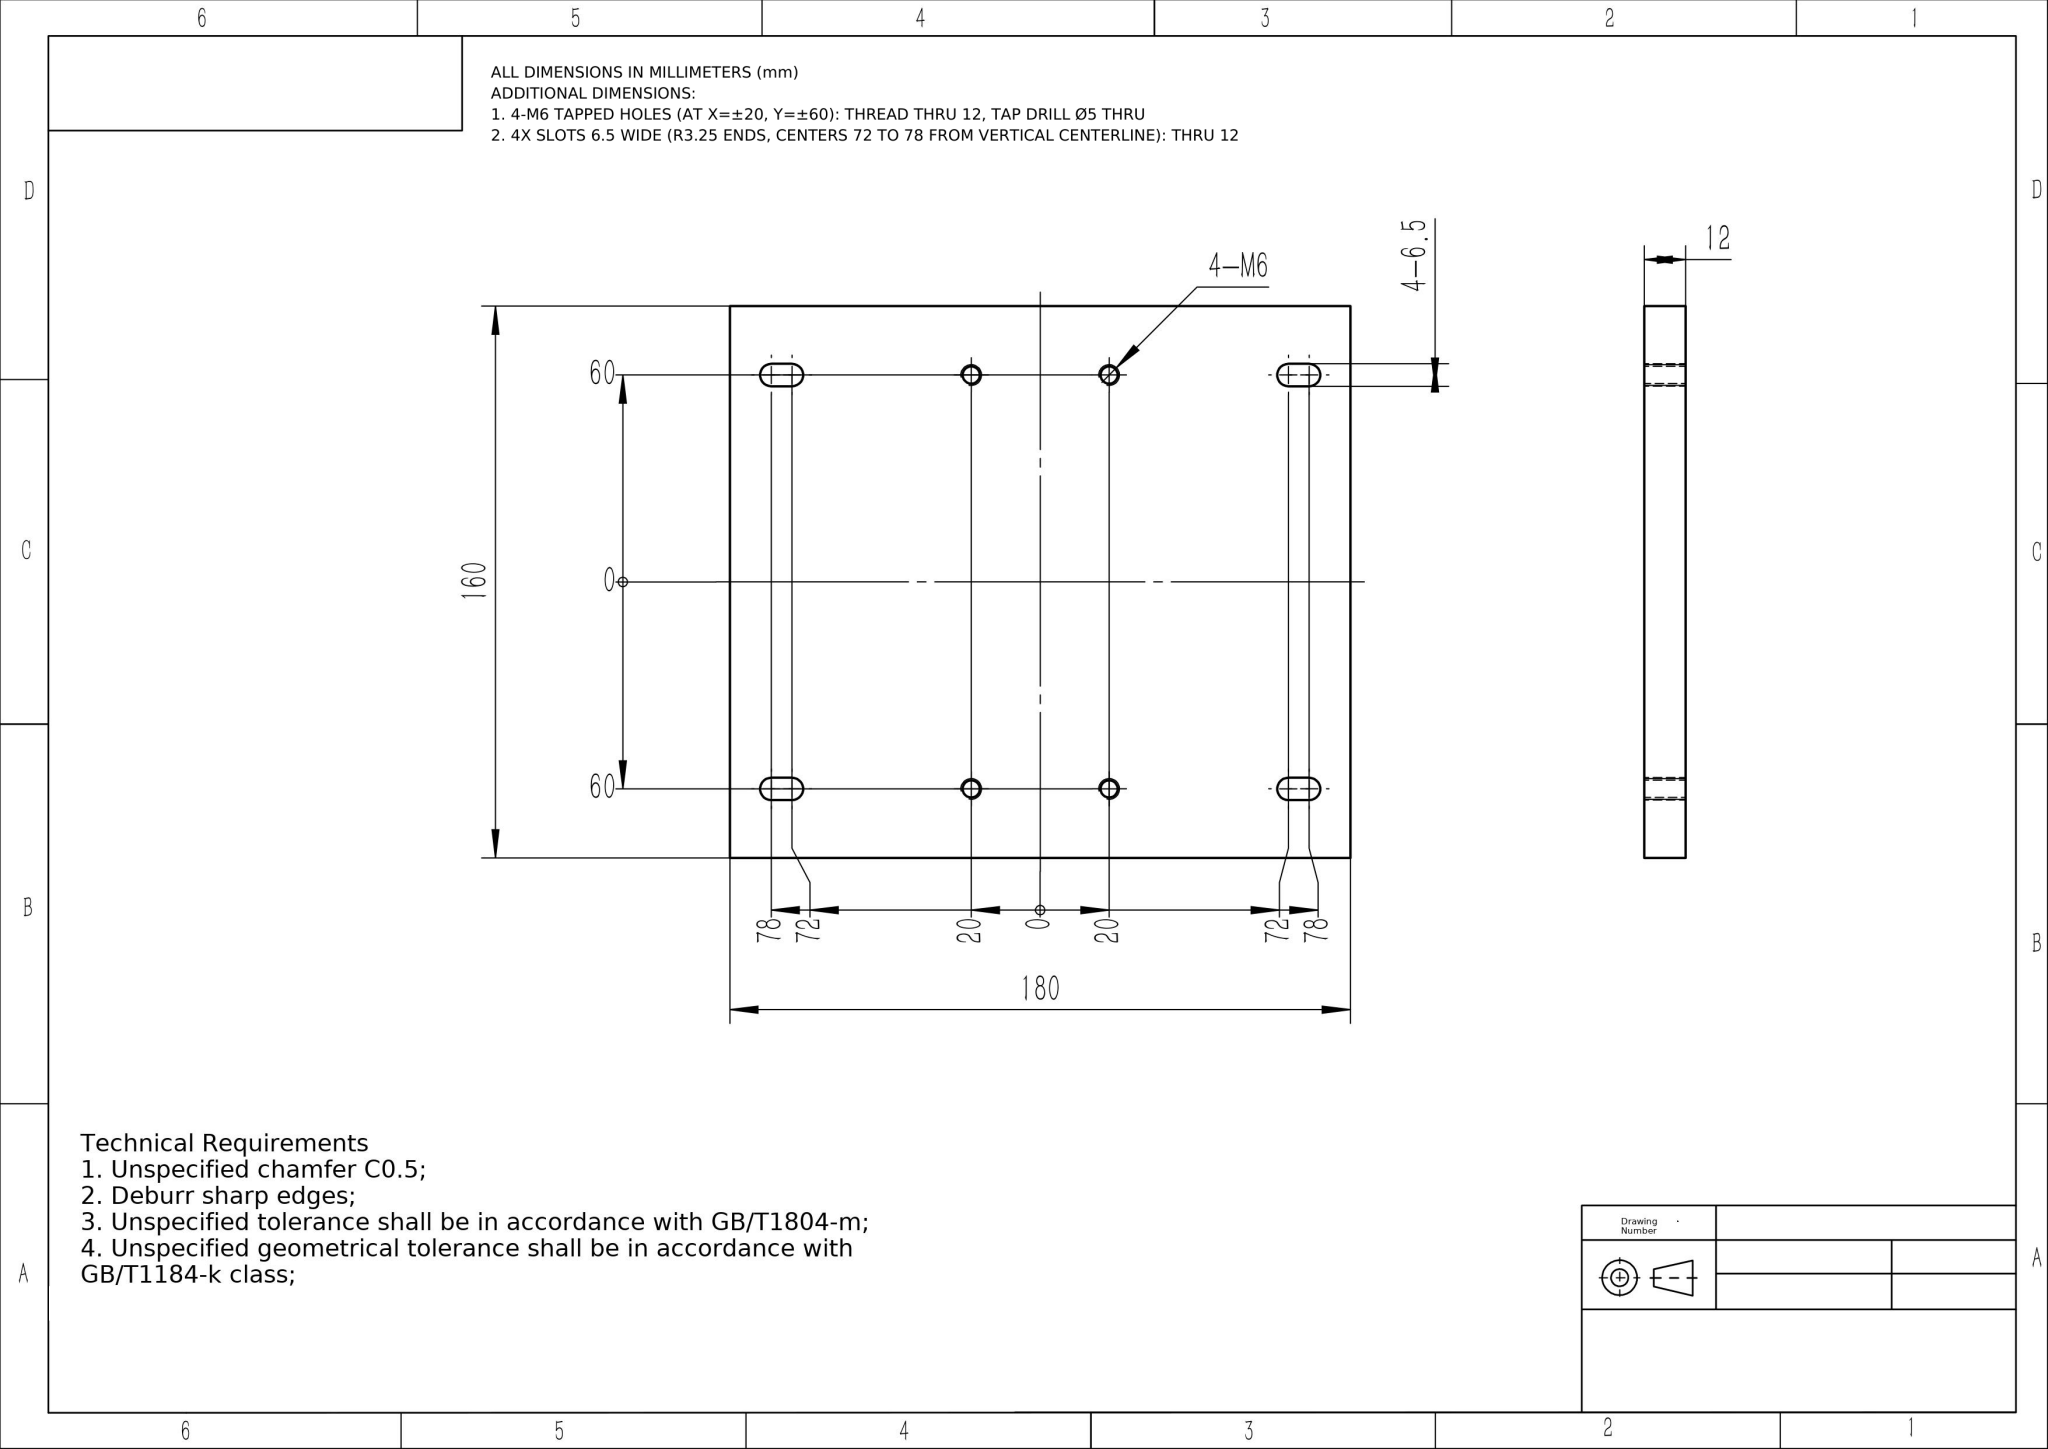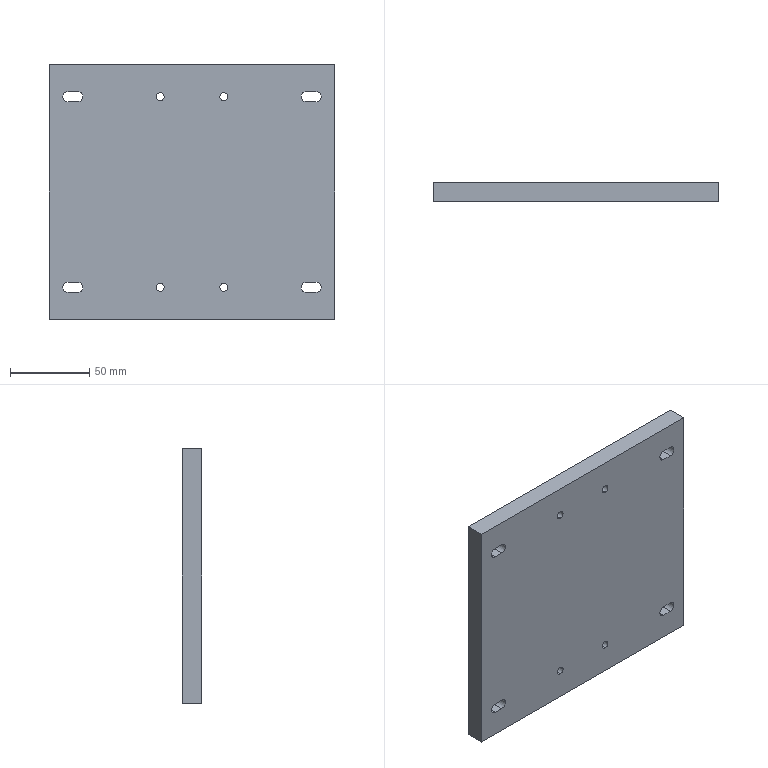Part | NX | mm | 1 solid | 30 faces | box 180 x 12 x 160 mm | volume 341193 mm3 | cylinder 16 | plane 14 | commonest cylinder face diameters 5 x8 6.5 x8